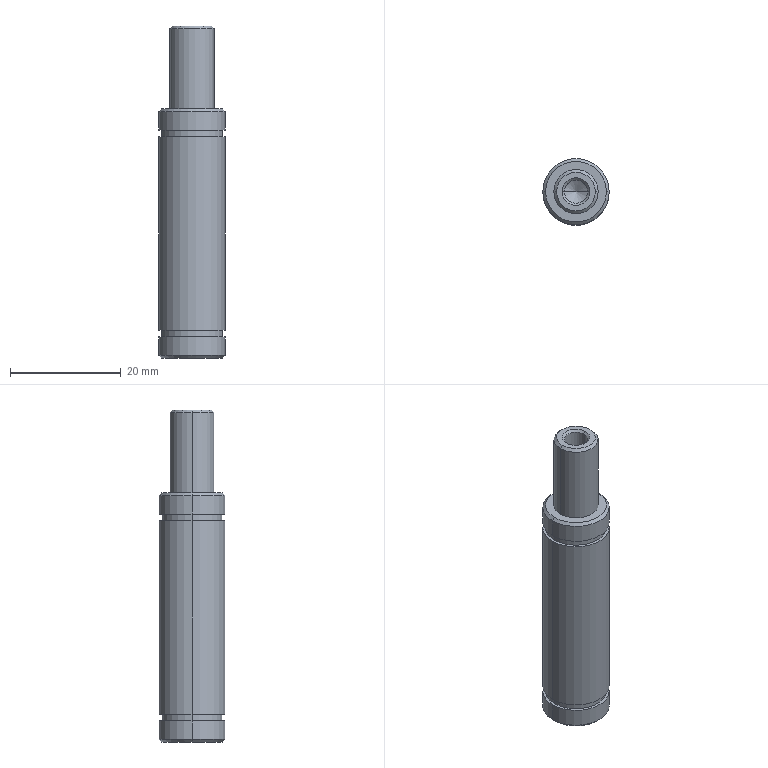Component | SolidWorks | GluePaperFeedingTensioningWheelAssembly-1_YX-04-118GluePaperFeedingTensioningWheelAxis-1 | 1 solid | 31 faces | box 12 x 12 x 60 mm | volume 5606 mm3 | cylinder 14 | cone 10 | plane 7 | commonest cylinder face diameters 12 x6 11 x4 8 x2 4.2 x2 | material 45#Steel
build123d program:
from build123d import *


with BuildPart() as part:
    # Sketch1 → Revolve1 (revolve)
    with BuildSketch(Plane.XY, mode=Mode.PRIVATE) as revolve1_sk:
        Polygon((12.6, 2.1), (13.862, 0), (60, 0), (60, 5.5), (59.5, 6), (56.2, 6), (56.2, 5.5), (55, 5.5), (55, 6), (20, 6), (20, 5.5), (18.8, 5.5), (18.8, 6), (15.5, 6), (15, 5.5), (15, 4), (0.5, 4), (0, 3.5), (0, 2.5), (0.4, 2.1), align=None)
    revolve(revolve1_sk.sketch.rotate(Axis((0, 0, 0), (1, 0, 0)), 270), axis=Axis((0, 0, 0), (1, 0, 0)))


solid = part.part

# Placed as in the assembly
solid = solid.moved(Location((16.603, 20.762, 174), (0, 90, 0)))
STEP:
#1=CARTESIAN_POINT('',(0.7363,0.8174,6.835));
#2=VERTEX_POINT('',#1);
#3=CARTESIAN_POINT('',(0.571,0.8174,6.835));
#4=VERTEX_POINT('',#3);
#5=CARTESIAN_POINT('',(0.6537,0.8174,6.835));
#6=DIRECTION('',(-0.,0.,-1.));
#7=DIRECTION('',(-1.,0.,0.));
#8=AXIS2_PLACEMENT_3D('',#5,#6,#7);
#9=CIRCLE('',#8,0.08268);
#10=EDGE_CURVE('',#2,#4,#9,.T.);
#11=ORIENTED_EDGE('',*,*,#10,.T.);
#12=CARTESIAN_POINT('',(0.5552,0.8174,6.85));
#13=VERTEX_POINT('',#12);
#14=CARTESIAN_POINT('',(0.5552,0.8174,6.85));
#15=DIRECTION('',(-0.7071,0.,0.7071));
#16=VECTOR('',#15,39.37);
#17=LINE('',#14,#16);
#18=EDGE_CURVE('',#4,#13,#17,.T.);
#19=ORIENTED_EDGE('',*,*,#18,.T.);
#20=CARTESIAN_POINT('',(0.7521,0.8174,6.85));
#21=VERTEX_POINT('',#20);
#22=CARTESIAN_POINT('',(0.6537,0.8174,6.85));
#23=DIRECTION('',(-0.,0.,-1.));
#24=DIRECTION('',(-1.,0.,0.));
#25=AXIS2_PLACEMENT_3D('',#22,#23,#24);
#26=CIRCLE('',#25,0.09843);
#27=EDGE_CURVE('',#21,#13,#26,.T.);
#28=ORIENTED_EDGE('',*,*,#27,.F.);
#29=CARTESIAN_POINT('',(0.7521,0.8174,6.85));
#30=DIRECTION('',(0.7071,0.,0.7071));
#31=VECTOR('',#30,39.37);
#32=LINE('',#29,#31);
#33=EDGE_CURVE('',#2,#21,#32,.T.);
#34=ORIENTED_EDGE('',*,*,#33,.F.);
#35=EDGE_LOOP('',(#11,#19,#28,#34));
#36=FACE_OUTER_BOUND('',#35,.T.);
#37=CARTESIAN_POINT('',(0.6537,0.8174,6.85));
#38=DIRECTION('',(0.,-0.,1.));
#39=DIRECTION('',(1.,0.,0.));
#40=AXIS2_PLACEMENT_3D('',#37,#38,#39);
#41=CONICAL_SURFACE('',#40,0.09843,0.7854);
#42=ADVANCED_FACE('',(#36),#41,.F.);
#43=CARTESIAN_POINT('',(0.5159,0.8174,6.85));
#44=VERTEX_POINT('',#43);
#45=CARTESIAN_POINT('',(0.7914,0.8174,6.85));
#46=VERTEX_POINT('',#45);
#47=CARTESIAN_POINT('',(0.6537,0.8174,6.85));
#48=DIRECTION('',(-0.,0.,-1.));
#49=DIRECTION('',(-1.,0.,0.));
#50=AXIS2_PLACEMENT_3D('',#47,#48,#49);
#51=CIRCLE('',#50,0.1378);
#52=EDGE_CURVE('',#44,#46,#51,.T.);
#53=ORIENTED_EDGE('',*,*,#52,.T.);
#54=CARTESIAN_POINT('',(0.8111,0.8174,6.831));
#55=VERTEX_POINT('',#54);
#56=CARTESIAN_POINT('',(0.8111,0.8174,6.831));
#57=DIRECTION('',(0.7071,0.,-0.7071));
#58=VECTOR('',#57,39.37);
#59=LINE('',#56,#58);
#60=EDGE_CURVE('',#46,#55,#59,.T.);
#61=ORIENTED_EDGE('',*,*,#60,.T.);
#62=CARTESIAN_POINT('',(0.4962,0.8174,6.831));
#63=VERTEX_POINT('',#62);
#64=CARTESIAN_POINT('',(0.6537,0.8174,6.831));
#65=DIRECTION('',(-0.,0.,-1.));
#66=DIRECTION('',(-1.,0.,0.));
#67=AXIS2_PLACEMENT_3D('',#64,#65,#66);
#68=CIRCLE('',#67,0.1575);
#69=EDGE_CURVE('',#63,#55,#68,.T.);
#70=ORIENTED_EDGE('',*,*,#69,.F.);
#71=CARTESIAN_POINT('',(0.4962,0.8174,6.831));
#72=DIRECTION('',(-0.7071,-0.,-0.7071));
#73=VECTOR('',#72,39.37);
#74=LINE('',#71,#73);
#75=EDGE_CURVE('',#44,#63,#74,.T.);
#76=ORIENTED_EDGE('',*,*,#75,.F.);
#77=EDGE_LOOP('',(#53,#61,#70,#76));
#78=FACE_OUTER_BOUND('',#77,.T.);
#79=CARTESIAN_POINT('',(0.6537,0.8174,6.831));
#80=DIRECTION('',(-0.,0.,-1.));
#81=DIRECTION('',(-1.,0.,0.));
#82=AXIS2_PLACEMENT_3D('',#79,#80,#81);
#83=CONICAL_SURFACE('',#82,0.1575,0.7854);
#84=ADVANCED_FACE('',(#78),#83,.T.);
#85=ORIENTED_EDGE('',*,*,#69,.T.);
#86=CARTESIAN_POINT('',(0.8111,0.8174,6.26));
#87=VERTEX_POINT('',#86);
#88=CARTESIAN_POINT('',(0.8111,0.8174,6.85));
#89=DIRECTION('',(-0.,0.,-1.));
#90=VECTOR('',#89,39.37);
#91=LINE('',#88,#90);
#92=EDGE_CURVE('',#55,#87,#91,.T.);
#93=ORIENTED_EDGE('',*,*,#92,.T.);
#94=CARTESIAN_POINT('',(0.4962,0.8174,6.26));
#95=VERTEX_POINT('',#94);
#96=CARTESIAN_POINT('',(0.6537,0.8174,6.26));
#97=DIRECTION('',(-0.,0.,-1.));
#98=DIRECTION('',(-1.,0.,0.));
#99=AXIS2_PLACEMENT_3D('',#96,#97,#98);
#100=CIRCLE('',#99,0.1575);
#101=EDGE_CURVE('',#95,#87,#100,.T.);
#102=ORIENTED_EDGE('',*,*,#101,.F.);
#103=CARTESIAN_POINT('',(0.4962,0.8174,6.85));
#104=DIRECTION('',(-0.,0.,-1.));
#105=VECTOR('',#104,39.37);
#106=LINE('',#103,#105);
#107=EDGE_CURVE('',#63,#95,#106,.T.);
#108=ORIENTED_EDGE('',*,*,#107,.F.);
#109=EDGE_LOOP('',(#85,#93,#102,#108));
#110=FACE_OUTER_BOUND('',#109,.T.);
#111=CARTESIAN_POINT('',(0.6537,0.8174,6.85));
#112=DIRECTION('',(-0.,0.,-1.));
#113=DIRECTION('',(-1.,0.,0.));
#114=AXIS2_PLACEMENT_3D('',#111,#112,#113);
#115=CYLINDRICAL_SURFACE('',#114,0.1575);
#116=ADVANCED_FACE('',(#110),#115,.T.);
#117=CARTESIAN_POINT('',(0.4371,0.8174,6.26));
#118=VERTEX_POINT('',#117);
#119=CARTESIAN_POINT('',(0.8702,0.8174,6.26));
#120=VERTEX_POINT('',#119);
#121=CARTESIAN_POINT('',(0.6537,0.8174,6.26));
#122=DIRECTION('',(-0.,0.,-1.));
#123=DIRECTION('',(-1.,0.,0.));
#124=AXIS2_PLACEMENT_3D('',#121,#122,#123);
#125=CIRCLE('',#124,0.2165);
#126=EDGE_CURVE('',#118,#120,#125,.T.);
#127=ORIENTED_EDGE('',*,*,#126,.T.);
#128=CARTESIAN_POINT('',(0.8899,0.8174,6.24));
#129=VERTEX_POINT('',#128);
#130=CARTESIAN_POINT('',(0.8899,0.8174,6.24));
#131=DIRECTION('',(0.7071,0.,-0.7071));
#132=VECTOR('',#131,39.37);
#133=LINE('',#130,#132);
#134=EDGE_CURVE('',#120,#129,#133,.T.);
#135=ORIENTED_EDGE('',*,*,#134,.T.);
#136=CARTESIAN_POINT('',(0.4174,0.8174,6.24));
#137=VERTEX_POINT('',#136);
#138=CARTESIAN_POINT('',(0.6537,0.8174,6.24));
#139=DIRECTION('',(-0.,0.,-1.));
#140=DIRECTION('',(-1.,0.,0.));
#141=AXIS2_PLACEMENT_3D('',#138,#139,#140);
#142=CIRCLE('',#141,0.2362);
#143=EDGE_CURVE('',#137,#129,#142,.T.);
#144=ORIENTED_EDGE('',*,*,#143,.F.);
#145=CARTESIAN_POINT('',(0.4174,0.8174,6.24));
#146=DIRECTION('',(-0.7071,-0.,-0.7071));
#147=VECTOR('',#146,39.37);
#148=LINE('',#145,#147);
#149=EDGE_CURVE('',#118,#137,#148,.T.);
#150=ORIENTED_EDGE('',*,*,#149,.F.);
#151=EDGE_LOOP('',(#127,#135,#144,#150));
#152=FACE_OUTER_BOUND('',#151,.T.);
#153=CARTESIAN_POINT('',(0.6537,0.8174,6.24));
#154=DIRECTION('',(-0.,0.,-1.));
#155=DIRECTION('',(-1.,0.,0.));
#156=AXIS2_PLACEMENT_3D('',#153,#154,#155);
#157=CONICAL_SURFACE('',#156,0.2362,0.7854);
#158=ADVANCED_FACE('',(#152),#157,.T.);
#159=ORIENTED_EDGE('',*,*,#143,.T.);
#160=CARTESIAN_POINT('',(0.8899,0.8174,6.11));
#161=VERTEX_POINT('',#160);
#162=CARTESIAN_POINT('',(0.8899,0.8174,6.85));
#163=DIRECTION('',(-0.,0.,-1.));
#164=VECTOR('',#163,39.37);
#165=LINE('',#162,#164);
#166=EDGE_CURVE('',#129,#161,#165,.T.);
#167=ORIENTED_EDGE('',*,*,#166,.T.);
#168=CARTESIAN_POINT('',(0.4174,0.8174,6.11));
#169=VERTEX_POINT('',#168);
#170=CARTESIAN_POINT('',(0.6537,0.8174,6.11));
#171=DIRECTION('',(-0.,0.,-1.));
#172=DIRECTION('',(-1.,0.,0.));
#173=AXIS2_PLACEMENT_3D('',#170,#171,#172);
#174=CIRCLE('',#173,0.2362);
#175=EDGE_CURVE('',#169,#161,#174,.T.);
#176=ORIENTED_EDGE('',*,*,#175,.F.);
#177=CARTESIAN_POINT('',(0.4174,0.8174,6.85));
#178=DIRECTION('',(-0.,0.,-1.));
#179=VECTOR('',#178,39.37);
#180=LINE('',#177,#179);
#181=EDGE_CURVE('',#137,#169,#180,.T.);
#182=ORIENTED_EDGE('',*,*,#181,.F.);
#183=EDGE_LOOP('',(#159,#167,#176,#182));
#184=FACE_OUTER_BOUND('',#183,.T.);
#185=CARTESIAN_POINT('',(0.6537,0.8174,6.85));
#186=DIRECTION('',(-0.,0.,-1.));
#187=DIRECTION('',(-1.,0.,0.));
#188=AXIS2_PLACEMENT_3D('',#185,#186,#187);
#189=CYLINDRICAL_SURFACE('',#188,0.2362);
#190=ADVANCED_FACE('',(#184),#189,.T.);
#191=CARTESIAN_POINT('',(0.4371,0.8174,6.11));
#192=VERTEX_POINT('',#191);
#193=CARTESIAN_POINT('',(0.8702,0.8174,6.11));
#194=VERTEX_POINT('',#193);
#195=CARTESIAN_POINT('',(0.6537,0.8174,6.11));
#196=DIRECTION('',(-0.,0.,-1.));
#197=DIRECTION('',(-1.,0.,0.));
#198=AXIS2_PLACEMENT_3D('',#195,#196,#197);
#199=CIRCLE('',#198,0.2165);
#200=EDGE_CURVE('',#192,#194,#199,.T.);
#201=ORIENTED_EDGE('',*,*,#200,.T.);
#202=CARTESIAN_POINT('',(0.8702,0.8174,6.063));
#203=VERTEX_POINT('',#202);
#204=CARTESIAN_POINT('',(0.8702,0.8174,6.85));
#205=DIRECTION('',(-0.,0.,-1.));
#206=VECTOR('',#205,39.37);
#207=LINE('',#204,#206);
#208=EDGE_CURVE('',#194,#203,#207,.T.);
#209=ORIENTED_EDGE('',*,*,#208,.T.);
#210=CARTESIAN_POINT('',(0.4371,0.8174,6.063));
#211=VERTEX_POINT('',#210);
#212=CARTESIAN_POINT('',(0.6537,0.8174,6.063));
#213=DIRECTION('',(-0.,0.,-1.));
#214=DIRECTION('',(-1.,0.,0.));
#215=AXIS2_PLACEMENT_3D('',#212,#213,#214);
#216=CIRCLE('',#215,0.2165);
#217=EDGE_CURVE('',#211,#203,#216,.T.);
#218=ORIENTED_EDGE('',*,*,#217,.F.);
#219=CARTESIAN_POINT('',(0.4371,0.8174,6.85));
#220=DIRECTION('',(-0.,0.,-1.));
#221=VECTOR('',#220,39.37);
#222=LINE('',#219,#221);
#223=EDGE_CURVE('',#192,#211,#222,.T.);
#224=ORIENTED_EDGE('',*,*,#223,.F.);
#225=EDGE_LOOP('',(#201,#209,#218,#224));
#226=FACE_OUTER_BOUND('',#225,.T.);
#227=CARTESIAN_POINT('',(0.6537,0.8174,6.85));
#228=DIRECTION('',(-0.,0.,-1.));
#229=DIRECTION('',(-1.,0.,0.));
#230=AXIS2_PLACEMENT_3D('',#227,#228,#229);
#231=CYLINDRICAL_SURFACE('',#230,0.2165);
#232=ADVANCED_FACE('',(#226),#231,.T.);
#233=CARTESIAN_POINT('',(0.4174,0.8174,6.063));
#234=VERTEX_POINT('',#233);
#235=CARTESIAN_POINT('',(0.8899,0.8174,6.063));
#236=VERTEX_POINT('',#235);
#237=CARTESIAN_POINT('',(0.6537,0.8174,6.063));
#238=DIRECTION('',(-0.,0.,-1.));
#239=DIRECTION('',(-1.,0.,0.));
#240=AXIS2_PLACEMENT_3D('',#237,#238,#239);
#241=CIRCLE('',#240,0.2362);
#242=EDGE_CURVE('',#234,#236,#241,.T.);
#243=ORIENTED_EDGE('',*,*,#242,.T.);
#244=CARTESIAN_POINT('',(0.8899,0.8174,4.685));
#245=VERTEX_POINT('',#244);
#246=CARTESIAN_POINT('',(0.8899,0.8174,6.85));
#247=DIRECTION('',(-0.,0.,-1.));
#248=VECTOR('',#247,39.37);
#249=LINE('',#246,#248);
#250=EDGE_CURVE('',#236,#245,#249,.T.);
#251=ORIENTED_EDGE('',*,*,#250,.T.);
#252=CARTESIAN_POINT('',(0.4174,0.8174,4.685));
#253=VERTEX_POINT('',#252);
#254=CARTESIAN_POINT('',(0.6537,0.8174,4.685));
#255=DIRECTION('',(-0.,0.,-1.));
#256=DIRECTION('',(-1.,0.,0.));
#257=AXIS2_PLACEMENT_3D('',#254,#255,#256);
#258=CIRCLE('',#257,0.2362);
#259=EDGE_CURVE('',#253,#245,#258,.T.);
#260=ORIENTED_EDGE('',*,*,#259,.F.);
#261=CARTESIAN_POINT('',(0.4174,0.8174,6.85));
#262=DIRECTION('',(-0.,0.,-1.));
#263=VECTOR('',#262,39.37);
#264=LINE('',#261,#263);
#265=EDGE_CURVE('',#234,#253,#264,.T.);
#266=ORIENTED_EDGE('',*,*,#265,.F.);
#267=EDGE_LOOP('',(#243,#251,#260,#266));
#268=FACE_OUTER_BOUND('',#267,.T.);
#269=CARTESIAN_POINT('',(0.6537,0.8174,6.85));
#270=DIRECTION('',(-0.,0.,-1.));
#271=DIRECTION('',(-1.,0.,0.));
#272=AXIS2_PLACEMENT_3D('',#269,#270,#271);
#273=CYLINDRICAL_SURFACE('',#272,0.2362);
#274=ADVANCED_FACE('',(#268),#273,.T.);
#275=CARTESIAN_POINT('',(0.4371,0.8174,4.685));
#276=VERTEX_POINT('',#275);
#277=CARTESIAN_POINT('',(0.8702,0.8174,4.685));
#278=VERTEX_POINT('',#277);
#279=CARTESIAN_POINT('',(0.6537,0.8174,4.685));
#280=DIRECTION('',(-0.,0.,-1.));
#281=DIRECTION('',(-1.,0.,0.));
#282=AXIS2_PLACEMENT_3D('',#279,#280,#281);
#283=CIRCLE('',#282,0.2165);
#284=EDGE_CURVE('',#276,#278,#283,.T.);
#285=ORIENTED_EDGE('',*,*,#284,.T.);
#286=CARTESIAN_POINT('',(0.8702,0.8174,4.638));
#287=VERTEX_POINT('',#286);
#288=CARTESIAN_POINT('',(0.8702,0.8174,6.85));
#289=DIRECTION('',(-0.,0.,-1.));
#290=VECTOR('',#289,39.37);
#291=LINE('',#288,#290);
#292=EDGE_CURVE('',#278,#287,#291,.T.);
#293=ORIENTED_EDGE('',*,*,#292,.T.);
#294=CARTESIAN_POINT('',(0.4371,0.8174,4.638));
#295=VERTEX_POINT('',#294);
#296=CARTESIAN_POINT('',(0.6537,0.8174,4.638));
#297=DIRECTION('',(-0.,0.,-1.));
#298=DIRECTION('',(-1.,0.,0.));
#299=AXIS2_PLACEMENT_3D('',#296,#297,#298);
#300=CIRCLE('',#299,0.2165);
#301=EDGE_CURVE('',#295,#287,#300,.T.);
#302=ORIENTED_EDGE('',*,*,#301,.F.);
#303=CARTESIAN_POINT('',(0.4371,0.8174,6.85));
#304=DIRECTION('',(-0.,0.,-1.));
#305=VECTOR('',#304,39.37);
#306=LINE('',#303,#305);
#307=EDGE_CURVE('',#276,#295,#306,.T.);
#308=ORIENTED_EDGE('',*,*,#307,.F.);
#309=EDGE_LOOP('',(#285,#293,#302,#308));
#310=FACE_OUTER_BOUND('',#309,.T.);
#311=CARTESIAN_POINT('',(0.6537,0.8174,6.85));
#312=DIRECTION('',(-0.,0.,-1.));
#313=DIRECTION('',(-1.,0.,0.));
#314=AXIS2_PLACEMENT_3D('',#311,#312,#313);
#315=CYLINDRICAL_SURFACE('',#314,0.2165);
#316=ADVANCED_FACE('',(#310),#315,.T.);
#317=CARTESIAN_POINT('',(0.4174,0.8174,4.638));
#318=VERTEX_POINT('',#317);
#319=CARTESIAN_POINT('',(0.8899,0.8174,4.638));
#320=VERTEX_POINT('',#319);
#321=CARTESIAN_POINT('',(0.6537,0.8174,4.638));
#322=DIRECTION('',(-0.,0.,-1.));
#323=DIRECTION('',(-1.,0.,0.));
#324=AXIS2_PLACEMENT_3D('',#321,#322,#323);
#325=CIRCLE('',#324,0.2362);
#326=EDGE_CURVE('',#318,#320,#325,.T.);
#327=ORIENTED_EDGE('',*,*,#326,.T.);
#328=CARTESIAN_POINT('',(0.8899,0.8174,4.508));
#329=VERTEX_POINT('',#328);
#330=CARTESIAN_POINT('',(0.8899,0.8174,6.85));
#331=DIRECTION('',(-0.,0.,-1.));
#332=VECTOR('',#331,39.37);
#333=LINE('',#330,#332);
#334=EDGE_CURVE('',#320,#329,#333,.T.);
#335=ORIENTED_EDGE('',*,*,#334,.T.);
#336=CARTESIAN_POINT('',(0.4174,0.8174,4.508));
#337=VERTEX_POINT('',#336);
#338=CARTESIAN_POINT('',(0.6537,0.8174,4.508));
#339=DIRECTION('',(-0.,0.,-1.));
#340=DIRECTION('',(-1.,0.,0.));
#341=AXIS2_PLACEMENT_3D('',#338,#339,#340);
#342=CIRCLE('',#341,0.2362);
#343=EDGE_CURVE('',#337,#329,#342,.T.);
#344=ORIENTED_EDGE('',*,*,#343,.F.);
#345=CARTESIAN_POINT('',(0.4174,0.8174,6.85));
#346=DIRECTION('',(-0.,0.,-1.));
#347=VECTOR('',#346,39.37);
#348=LINE('',#345,#347);
#349=EDGE_CURVE('',#318,#337,#348,.T.);
#350=ORIENTED_EDGE('',*,*,#349,.F.);
#351=EDGE_LOOP('',(#327,#335,#344,#350));
#352=FACE_OUTER_BOUND('',#351,.T.);
#353=CARTESIAN_POINT('',(0.6537,0.8174,6.85));
#354=DIRECTION('',(-0.,0.,-1.));
#355=DIRECTION('',(-1.,0.,0.));
#356=AXIS2_PLACEMENT_3D('',#353,#354,#355);
#357=CYLINDRICAL_SURFACE('',#356,0.2362);
#358=ADVANCED_FACE('',(#352),#357,.T.);
#359=CARTESIAN_POINT('',(0.4371,0.8174,4.488));
#360=VERTEX_POINT('',#359);
#361=CARTESIAN_POINT('',(0.8702,0.8174,4.488));
#362=VERTEX_POINT('',#361);
#363=CARTESIAN_POINT('',(0.6537,0.8174,4.488));
#364=DIRECTION('',(-0.,0.,-1.));
#365=DIRECTION('',(-1.,0.,0.));
#366=AXIS2_PLACEMENT_3D('',#363,#364,#365);
#367=CIRCLE('',#366,0.2165);
#368=EDGE_CURVE('',#360,#362,#367,.T.);
#369=ORIENTED_EDGE('',*,*,#368,.F.);
#370=CARTESIAN_POINT('',(0.4371,0.8174,4.488));
#371=DIRECTION('',(-0.7071,0.,0.7071));
#372=VECTOR('',#371,39.37);
#373=LINE('',#370,#372);
#374=EDGE_CURVE('',#360,#337,#373,.T.);
#375=ORIENTED_EDGE('',*,*,#374,.T.);
#376=ORIENTED_EDGE('',*,*,#343,.T.);
#377=CARTESIAN_POINT('',(0.8702,0.8174,4.488));
#378=DIRECTION('',(0.7071,0.,0.7071));
#379=VECTOR('',#378,39.37);
#380=LINE('',#377,#379);
#381=EDGE_CURVE('',#362,#329,#380,.T.);
#382=ORIENTED_EDGE('',*,*,#381,.F.);
#383=EDGE_LOOP('',(#369,#375,#376,#382));
#384=FACE_OUTER_BOUND('',#383,.T.);
#385=CARTESIAN_POINT('',(0.6537,0.8174,4.488));
#386=DIRECTION('',(0.,-0.,1.));
#387=DIRECTION('',(1.,0.,0.));
#388=AXIS2_PLACEMENT_3D('',#385,#386,#387);
#389=CONICAL_SURFACE('',#388,0.2165,0.7854);
#390=ADVANCED_FACE('',(#384),#389,.T.);
#391=CARTESIAN_POINT('',(0.6537,0.8174,6.305));
#392=VERTEX_POINT('',#391);
#393=CARTESIAN_POINT('',(0.7363,0.8174,6.354));
#394=VERTEX_POINT('',#393);
#395=CARTESIAN_POINT('',(0.7363,0.8174,6.354));
#396=DIRECTION('',(0.8572,0.,0.515));
#397=VECTOR('',#396,39.37);
#398=LINE('',#395,#397);
#399=EDGE_CURVE('',#392,#394,#398,.T.);
#400=ORIENTED_EDGE('',*,*,#399,.F.);
#401=CARTESIAN_POINT('',(0.571,0.8174,6.354));
#402=VERTEX_POINT('',#401);
#403=CARTESIAN_POINT('',(0.571,0.8174,6.354));
#404=DIRECTION('',(-0.8572,0.,0.515));
#405=VECTOR('',#404,39.37);
#406=LINE('',#403,#405);
#407=EDGE_CURVE('',#392,#402,#406,.T.);
#408=ORIENTED_EDGE('',*,*,#407,.T.);
#409=CARTESIAN_POINT('',(0.6537,0.8174,6.354));
#410=DIRECTION('',(-0.,0.,-1.));
#411=DIRECTION('',(-1.,0.,0.));
#412=AXIS2_PLACEMENT_3D('',#409,#410,#411);
#413=CIRCLE('',#412,0.08268);
#414=EDGE_CURVE('',#394,#402,#413,.T.);
#415=ORIENTED_EDGE('',*,*,#414,.F.);
#416=EDGE_LOOP('',(#400,#408,#415));
#417=FACE_OUTER_BOUND('',#416,.T.);
#418=CARTESIAN_POINT('',(0.6537,0.8174,6.354));
#419=DIRECTION('',(0.,-0.,1.));
#420=DIRECTION('',(1.,0.,0.));
#421=AXIS2_PLACEMENT_3D('',#418,#419,#420);
#422=CONICAL_SURFACE('',#421,0.08268,1.03);
#423=ADVANCED_FACE('',(#417),#422,.F.);
#424=ORIENTED_EDGE('',*,*,#10,.F.);
#425=CARTESIAN_POINT('',(0.7363,0.8174,6.85));
#426=DIRECTION('',(-0.,0.,-1.));
#427=VECTOR('',#426,39.37);
#428=LINE('',#425,#427);
#429=EDGE_CURVE('',#2,#394,#428,.T.);
#430=ORIENTED_EDGE('',*,*,#429,.T.);
#431=ORIENTED_EDGE('',*,*,#414,.T.);
#432=CARTESIAN_POINT('',(0.571,0.8174,6.85));
#433=DIRECTION('',(-0.,0.,-1.));
#434=VECTOR('',#433,39.37);
#435=LINE('',#432,#434);
#436=EDGE_CURVE('',#4,#402,#435,.T.);
#437=ORIENTED_EDGE('',*,*,#436,.F.);
#438=EDGE_LOOP('',(#424,#430,#431,#437));
#439=FACE_OUTER_BOUND('',#438,.T.);
#440=CARTESIAN_POINT('',(0.6537,0.8174,6.85));
#441=DIRECTION('',(-0.,0.,-1.));
#442=DIRECTION('',(-1.,0.,0.));
#443=AXIS2_PLACEMENT_3D('',#440,#441,#442);
#444=CYLINDRICAL_SURFACE('',#443,0.08268);
#445=ADVANCED_FACE('',(#439),#444,.F.);
#446=ORIENTED_EDGE('',*,*,#429,.F.);
#447=CARTESIAN_POINT('',(0.6537,0.8174,6.835));
#448=DIRECTION('',(-0.,0.,-1.));
#449=DIRECTION('',(-1.,0.,0.));
#450=AXIS2_PLACEMENT_3D('',#447,#448,#449);
#451=CIRCLE('',#450,0.08268);
#452=EDGE_CURVE('',#4,#2,#451,.T.);
#453=ORIENTED_EDGE('',*,*,#452,.F.);
#454=ORIENTED_EDGE('',*,*,#436,.T.);
#455=CARTESIAN_POINT('',(0.6537,0.8174,6.354));
#456=DIRECTION('',(-0.,0.,-1.));
#457=DIRECTION('',(-1.,0.,0.));
#458=AXIS2_PLACEMENT_3D('',#455,#456,#457);
#459=CIRCLE('',#458,0.08268);
#460=EDGE_CURVE('',#402,#394,#459,.T.);
#461=ORIENTED_EDGE('',*,*,#460,.T.);
#462=EDGE_LOOP('',(#446,#453,#454,#461));
#463=FACE_OUTER_BOUND('',#462,.T.);
#464=CARTESIAN_POINT('',(0.6537,0.8174,6.85));
#465=DIRECTION('',(-0.,0.,-1.));
#466=DIRECTION('',(-1.,0.,0.));
#467=AXIS2_PLACEMENT_3D('',#464,#465,#466);
#468=CYLINDRICAL_SURFACE('',#467,0.08268);
#469=ADVANCED_FACE('',(#463),#468,.F.);
#470=ORIENTED_EDGE('',*,*,#407,.F.);
#471=ORIENTED_EDGE('',*,*,#399,.T.);
#472=ORIENTED_EDGE('',*,*,#460,.F.);
#473=EDGE_LOOP('',(#470,#471,#472));
#474=FACE_OUTER_BOUND('',#473,.T.);
#475=CARTESIAN_POINT('',(0.6537,0.8174,6.354));
#476=DIRECTION('',(0.,-0.,1.));
#477=DIRECTION('',(1.,0.,0.));
#478=AXIS2_PLACEMENT_3D('',#475,#476,#477);
#479=CONICAL_SURFACE('',#478,0.08268,1.03);
#480=ADVANCED_FACE('',(#474),#479,.F.);
#481=CARTESIAN_POINT('',(0.6537,0.8174,4.488));
#482=DIRECTION('',(-0.,0.,-1.));
#483=DIRECTION('',(-1.,0.,0.));
#484=AXIS2_PLACEMENT_3D('',#481,#482,#483);
#485=CIRCLE('',#484,0.2165);
#486=EDGE_CURVE('',#362,#360,#485,.T.);
#487=ORIENTED_EDGE('',*,*,#486,.T.);
#488=ORIENTED_EDGE('',*,*,#368,.T.);
#489=EDGE_LOOP('',(#487,#488));
#490=FACE_OUTER_BOUND('',#489,.T.);
#491=CARTESIAN_POINT('',(0.6537,0.8174,4.488));
#492=DIRECTION('',(-0.,0.,-1.));
#493=DIRECTION('',(-1.,-0.,0.));
#494=AXIS2_PLACEMENT_3D('',#491,#492,#493);
#495=PLANE('',#494);
#496=ADVANCED_FACE('',(#490),#495,.T.);
#497=ORIENTED_EDGE('',*,*,#374,.F.);
#498=ORIENTED_EDGE('',*,*,#486,.F.);
#499=ORIENTED_EDGE('',*,*,#381,.T.);
#500=CARTESIAN_POINT('',(0.6537,0.8174,4.508));
#501=DIRECTION('',(-0.,0.,-1.));
#502=DIRECTION('',(-1.,0.,0.));
#503=AXIS2_PLACEMENT_3D('',#500,#501,#502);
#504=CIRCLE('',#503,0.2362);
#505=EDGE_CURVE('',#329,#337,#504,.T.);
#506=ORIENTED_EDGE('',*,*,#505,.T.);
#507=EDGE_LOOP('',(#497,#498,#499,#506));
#508=FACE_OUTER_BOUND('',#507,.T.);
#509=CARTESIAN_POINT('',(0.6537,0.8174,4.488));
#510=DIRECTION('',(0.,-0.,1.));
#511=DIRECTION('',(1.,0.,0.));
#512=AXIS2_PLACEMENT_3D('',#509,#510,#511);
#513=CONICAL_SURFACE('',#512,0.2165,0.7854);
#514=ADVANCED_FACE('',(#508),#513,.T.);
#515=ORIENTED_EDGE('',*,*,#334,.F.);
#516=CARTESIAN_POINT('',(0.6537,0.8174,4.638));
#517=DIRECTION('',(-0.,0.,-1.));
#518=DIRECTION('',(-1.,0.,0.));
#519=AXIS2_PLACEMENT_3D('',#516,#517,#518);
#520=CIRCLE('',#519,0.2362);
#521=EDGE_CURVE('',#320,#318,#520,.T.);
#522=ORIENTED_EDGE('',*,*,#521,.T.);
#523=ORIENTED_EDGE('',*,*,#349,.T.);
#524=ORIENTED_EDGE('',*,*,#505,.F.);
#525=EDGE_LOOP('',(#515,#522,#523,#524));
#526=FACE_OUTER_BOUND('',#525,.T.);
#527=CARTESIAN_POINT('',(0.6537,0.8174,6.85));
#528=DIRECTION('',(-0.,0.,-1.));
#529=DIRECTION('',(-1.,0.,0.));
#530=AXIS2_PLACEMENT_3D('',#527,#528,#529);
#531=CYLINDRICAL_SURFACE('',#530,0.2362);
#532=ADVANCED_FACE('',(#526),#531,.T.);
#533=ORIENTED_EDGE('',*,*,#301,.T.);
#534=CARTESIAN_POINT('',(0.6537,0.8174,4.638));
#535=DIRECTION('',(-0.,0.,-1.));
#536=DIRECTION('',(-1.,0.,0.));
#537=AXIS2_PLACEMENT_3D('',#534,#535,#536);
#538=CIRCLE('',#537,0.2165);
#539=EDGE_CURVE('',#287,#295,#538,.T.);
#540=ORIENTED_EDGE('',*,*,#539,.T.);
#541=EDGE_LOOP('',(#533,#540));
#542=FACE_BOUND('',#541,.T.);
#543=ORIENTED_EDGE('',*,*,#326,.F.);
#544=ORIENTED_EDGE('',*,*,#521,.F.);
#545=EDGE_LOOP('',(#543,#544));
#546=FACE_OUTER_BOUND('',#545,.T.);
#547=CARTESIAN_POINT('',(0.6537,1.054,4.638));
#548=DIRECTION('',(0.,-0.,1.));
#549=DIRECTION('',(1.,0.,-0.));
#550=AXIS2_PLACEMENT_3D('',#547,#548,#549);
#551=PLANE('',#550);
#552=ADVANCED_FACE('',(#542,#546),#551,.T.);
#553=ORIENTED_EDGE('',*,*,#292,.F.);
#554=CARTESIAN_POINT('',(0.6537,0.8174,4.685));
#555=DIRECTION('',(-0.,0.,-1.));
#556=DIRECTION('',(-1.,0.,0.));
#557=AXIS2_PLACEMENT_3D('',#554,#555,#556);
#558=CIRCLE('',#557,0.2165);
#559=EDGE_CURVE('',#278,#276,#558,.T.);
#560=ORIENTED_EDGE('',*,*,#559,.T.);
#561=ORIENTED_EDGE('',*,*,#307,.T.);
#562=ORIENTED_EDGE('',*,*,#539,.F.);
#563=EDGE_LOOP('',(#553,#560,#561,#562));
#564=FACE_OUTER_BOUND('',#563,.T.);
#565=CARTESIAN_POINT('',(0.6537,0.8174,6.85));
#566=DIRECTION('',(-0.,0.,-1.));
#567=DIRECTION('',(-1.,0.,0.));
#568=AXIS2_PLACEMENT_3D('',#565,#566,#567);
#569=CYLINDRICAL_SURFACE('',#568,0.2165);
#570=ADVANCED_FACE('',(#564),#569,.T.);
#571=ORIENTED_EDGE('',*,*,#259,.T.);
#572=CARTESIAN_POINT('',(0.6537,0.8174,4.685));
#573=DIRECTION('',(-0.,0.,-1.));
#574=DIRECTION('',(-1.,0.,0.));
#575=AXIS2_PLACEMENT_3D('',#572,#573,#574);
#576=CIRCLE('',#575,0.2362);
#577=EDGE_CURVE('',#245,#253,#576,.T.);
#578=ORIENTED_EDGE('',*,*,#577,.T.);
#579=EDGE_LOOP('',(#571,#578));
#580=FACE_OUTER_BOUND('',#579,.T.);
#581=ORIENTED_EDGE('',*,*,#284,.F.);
#582=ORIENTED_EDGE('',*,*,#559,.F.);
#583=EDGE_LOOP('',(#581,#582));
#584=FACE_BOUND('',#583,.T.);
#585=CARTESIAN_POINT('',(0.6537,1.034,4.685));
#586=DIRECTION('',(-0.,0.,-1.));
#587=DIRECTION('',(-1.,-0.,0.));
#588=AXIS2_PLACEMENT_3D('',#585,#586,#587);
#589=PLANE('',#588);
#590=ADVANCED_FACE('',(#580,#584),#589,.T.);
#591=ORIENTED_EDGE('',*,*,#250,.F.);
#592=CARTESIAN_POINT('',(0.6537,0.8174,6.063));
#593=DIRECTION('',(-0.,0.,-1.));
#594=DIRECTION('',(-1.,0.,0.));
#595=AXIS2_PLACEMENT_3D('',#592,#593,#594);
#596=CIRCLE('',#595,0.2362);
#597=EDGE_CURVE('',#236,#234,#596,.T.);
#598=ORIENTED_EDGE('',*,*,#597,.T.);
#599=ORIENTED_EDGE('',*,*,#265,.T.);
#600=ORIENTED_EDGE('',*,*,#577,.F.);
#601=EDGE_LOOP('',(#591,#598,#599,#600));
#602=FACE_OUTER_BOUND('',#601,.T.);
#603=CARTESIAN_POINT('',(0.6537,0.8174,6.85));
#604=DIRECTION('',(-0.,0.,-1.));
#605=DIRECTION('',(-1.,0.,0.));
#606=AXIS2_PLACEMENT_3D('',#603,#604,#605);
#607=CYLINDRICAL_SURFACE('',#606,0.2362);
#608=ADVANCED_FACE('',(#602),#607,.T.);
#609=ORIENTED_EDGE('',*,*,#217,.T.);
#610=CARTESIAN_POINT('',(0.6537,0.8174,6.063));
#611=DIRECTION('',(-0.,0.,-1.));
#612=DIRECTION('',(-1.,0.,0.));
#613=AXIS2_PLACEMENT_3D('',#610,#611,#612);
#614=CIRCLE('',#613,0.2165);
#615=EDGE_CURVE('',#203,#211,#614,.T.);
#616=ORIENTED_EDGE('',*,*,#615,.T.);
#617=EDGE_LOOP('',(#609,#616));
#618=FACE_BOUND('',#617,.T.);
#619=ORIENTED_EDGE('',*,*,#242,.F.);
#620=ORIENTED_EDGE('',*,*,#597,.F.);
#621=EDGE_LOOP('',(#619,#620));
#622=FACE_OUTER_BOUND('',#621,.T.);
#623=CARTESIAN_POINT('',(0.6537,1.054,6.063));
#624=DIRECTION('',(0.,-0.,1.));
#625=DIRECTION('',(1.,0.,-0.));
#626=AXIS2_PLACEMENT_3D('',#623,#624,#625);
#627=PLANE('',#626);
#628=ADVANCED_FACE('',(#618,#622),#627,.T.);
#629=ORIENTED_EDGE('',*,*,#208,.F.);
#630=CARTESIAN_POINT('',(0.6537,0.8174,6.11));
#631=DIRECTION('',(-0.,0.,-1.));
#632=DIRECTION('',(-1.,0.,0.));
#633=AXIS2_PLACEMENT_3D('',#630,#631,#632);
#634=CIRCLE('',#633,0.2165);
#635=EDGE_CURVE('',#194,#192,#634,.T.);
#636=ORIENTED_EDGE('',*,*,#635,.T.);
#637=ORIENTED_EDGE('',*,*,#223,.T.);
#638=ORIENTED_EDGE('',*,*,#615,.F.);
#639=EDGE_LOOP('',(#629,#636,#637,#638));
#640=FACE_OUTER_BOUND('',#639,.T.);
#641=CARTESIAN_POINT('',(0.6537,0.8174,6.85));
#642=DIRECTION('',(-0.,0.,-1.));
#643=DIRECTION('',(-1.,0.,0.));
#644=AXIS2_PLACEMENT_3D('',#641,#642,#643);
#645=CYLINDRICAL_SURFACE('',#644,0.2165);
#646=ADVANCED_FACE('',(#640),#645,.T.);
#647=ORIENTED_EDGE('',*,*,#175,.T.);
#648=CARTESIAN_POINT('',(0.6537,0.8174,6.11));
#649=DIRECTION('',(-0.,0.,-1.));
#650=DIRECTION('',(-1.,0.,0.));
#651=AXIS2_PLACEMENT_3D('',#648,#649,#650);
#652=CIRCLE('',#651,0.2362);
#653=EDGE_CURVE('',#161,#169,#652,.T.);
#654=ORIENTED_EDGE('',*,*,#653,.T.);
#655=EDGE_LOOP('',(#647,#654));
#656=FACE_OUTER_BOUND('',#655,.T.);
#657=ORIENTED_EDGE('',*,*,#200,.F.);
#658=ORIENTED_EDGE('',*,*,#635,.F.);
#659=EDGE_LOOP('',(#657,#658));
#660=FACE_BOUND('',#659,.T.);
#661=CARTESIAN_POINT('',(0.6537,1.034,6.11));
#662=DIRECTION('',(-0.,0.,-1.));
#663=DIRECTION('',(-1.,-0.,0.));
#664=AXIS2_PLACEMENT_3D('',#661,#662,#663);
#665=PLANE('',#664);
#666=ADVANCED_FACE('',(#656,#660),#665,.T.);
#667=ORIENTED_EDGE('',*,*,#166,.F.);
#668=CARTESIAN_POINT('',(0.6537,0.8174,6.24));
#669=DIRECTION('',(-0.,0.,-1.));
#670=DIRECTION('',(-1.,0.,0.));
#671=AXIS2_PLACEMENT_3D('',#668,#669,#670);
#672=CIRCLE('',#671,0.2362);
#673=EDGE_CURVE('',#129,#137,#672,.T.);
#674=ORIENTED_EDGE('',*,*,#673,.T.);
#675=ORIENTED_EDGE('',*,*,#181,.T.);
#676=ORIENTED_EDGE('',*,*,#653,.F.);
#677=EDGE_LOOP('',(#667,#674,#675,#676));
#678=FACE_OUTER_BOUND('',#677,.T.);
#679=CARTESIAN_POINT('',(0.6537,0.8174,6.85));
#680=DIRECTION('',(-0.,0.,-1.));
#681=DIRECTION('',(-1.,0.,0.));
#682=AXIS2_PLACEMENT_3D('',#679,#680,#681);
#683=CYLINDRICAL_SURFACE('',#682,0.2362);
#684=ADVANCED_FACE('',(#678),#683,.T.);
#685=ORIENTED_EDGE('',*,*,#134,.F.);
#686=CARTESIAN_POINT('',(0.6537,0.8174,6.26));
#687=DIRECTION('',(-0.,0.,-1.));
#688=DIRECTION('',(-1.,0.,0.));
#689=AXIS2_PLACEMENT_3D('',#686,#687,#688);
#690=CIRCLE('',#689,0.2165);
#691=EDGE_CURVE('',#120,#118,#690,.T.);
#692=ORIENTED_EDGE('',*,*,#691,.T.);
#693=ORIENTED_EDGE('',*,*,#149,.T.);
#694=ORIENTED_EDGE('',*,*,#673,.F.);
#695=EDGE_LOOP('',(#685,#692,#693,#694));
#696=FACE_OUTER_BOUND('',#695,.T.);
#697=CARTESIAN_POINT('',(0.6537,0.8174,6.24));
#698=DIRECTION('',(-0.,0.,-1.));
#699=DIRECTION('',(-1.,0.,0.));
#700=AXIS2_PLACEMENT_3D('',#697,#698,#699);
#701=CONICAL_SURFACE('',#700,0.2362,0.7854);
#702=ADVANCED_FACE('',(#696),#701,.T.);
#703=ORIENTED_EDGE('',*,*,#101,.T.);
#704=CARTESIAN_POINT('',(0.6537,0.8174,6.26));
#705=DIRECTION('',(-0.,0.,-1.));
#706=DIRECTION('',(-1.,0.,0.));
#707=AXIS2_PLACEMENT_3D('',#704,#705,#706);
#708=CIRCLE('',#707,0.1575);
#709=EDGE_CURVE('',#87,#95,#708,.T.);
#710=ORIENTED_EDGE('',*,*,#709,.T.);
#711=EDGE_LOOP('',(#703,#710));
#712=FACE_BOUND('',#711,.T.);
#713=ORIENTED_EDGE('',*,*,#126,.F.);
#714=ORIENTED_EDGE('',*,*,#691,.F.);
#715=EDGE_LOOP('',(#713,#714));
#716=FACE_OUTER_BOUND('',#715,.T.);
#717=CARTESIAN_POINT('',(0.6537,1.034,6.26));
#718=DIRECTION('',(0.,-0.,1.));
#719=DIRECTION('',(1.,0.,-0.));
#720=AXIS2_PLACEMENT_3D('',#717,#718,#719);
#721=PLANE('',#720);
#722=ADVANCED_FACE('',(#712,#716),#721,.T.);
#723=ORIENTED_EDGE('',*,*,#92,.F.);
#724=CARTESIAN_POINT('',(0.6537,0.8174,6.831));
#725=DIRECTION('',(-0.,0.,-1.));
#726=DIRECTION('',(-1.,0.,0.));
#727=AXIS2_PLACEMENT_3D('',#724,#725,#726);
#728=CIRCLE('',#727,0.1575);
#729=EDGE_CURVE('',#55,#63,#728,.T.);
#730=ORIENTED_EDGE('',*,*,#729,.T.);
#731=ORIENTED_EDGE('',*,*,#107,.T.);
#732=ORIENTED_EDGE('',*,*,#709,.F.);
#733=EDGE_LOOP('',(#723,#730,#731,#732));
#734=FACE_OUTER_BOUND('',#733,.T.);
#735=CARTESIAN_POINT('',(0.6537,0.8174,6.85));
#736=DIRECTION('',(-0.,0.,-1.));
#737=DIRECTION('',(-1.,0.,0.));
#738=AXIS2_PLACEMENT_3D('',#735,#736,#737);
#739=CYLINDRICAL_SURFACE('',#738,0.1575);
#740=ADVANCED_FACE('',(#734),#739,.T.);
#741=ORIENTED_EDGE('',*,*,#60,.F.);
#742=CARTESIAN_POINT('',(0.6537,0.8174,6.85));
#743=DIRECTION('',(-0.,0.,-1.));
#744=DIRECTION('',(-1.,0.,0.));
#745=AXIS2_PLACEMENT_3D('',#742,#743,#744);
#746=CIRCLE('',#745,0.1378);
#747=EDGE_CURVE('',#46,#44,#746,.T.);
#748=ORIENTED_EDGE('',*,*,#747,.T.);
#749=ORIENTED_EDGE('',*,*,#75,.T.);
#750=ORIENTED_EDGE('',*,*,#729,.F.);
#751=EDGE_LOOP('',(#741,#748,#749,#750));
#752=FACE_OUTER_BOUND('',#751,.T.);
#753=CARTESIAN_POINT('',(0.6537,0.8174,6.831));
#754=DIRECTION('',(-0.,0.,-1.));
#755=DIRECTION('',(-1.,0.,0.));
#756=AXIS2_PLACEMENT_3D('',#753,#754,#755);
#757=CONICAL_SURFACE('',#756,0.1575,0.7854);
#758=ADVANCED_FACE('',(#752),#757,.T.);
#759=ORIENTED_EDGE('',*,*,#27,.T.);
#760=CARTESIAN_POINT('',(0.6537,0.8174,6.85));
#761=DIRECTION('',(-0.,0.,-1.));
#762=DIRECTION('',(-1.,0.,0.));
#763=AXIS2_PLACEMENT_3D('',#760,#761,#762);
#764=CIRCLE('',#763,0.09843);
#765=EDGE_CURVE('',#13,#21,#764,.T.);
#766=ORIENTED_EDGE('',*,*,#765,.T.);
#767=EDGE_LOOP('',(#759,#766));
#768=FACE_BOUND('',#767,.T.);
#769=ORIENTED_EDGE('',*,*,#52,.F.);
#770=ORIENTED_EDGE('',*,*,#747,.F.);
#771=EDGE_LOOP('',(#769,#770));
#772=FACE_OUTER_BOUND('',#771,.T.);
#773=CARTESIAN_POINT('',(0.6537,0.9552,6.85));
#774=DIRECTION('',(0.,-0.,1.));
#775=DIRECTION('',(1.,0.,-0.));
#776=AXIS2_PLACEMENT_3D('',#773,#774,#775);
#777=PLANE('',#776);
#778=ADVANCED_FACE('',(#768,#772),#777,.T.);
#779=ORIENTED_EDGE('',*,*,#18,.F.);
#780=ORIENTED_EDGE('',*,*,#452,.T.);
#781=ORIENTED_EDGE('',*,*,#33,.T.);
#782=ORIENTED_EDGE('',*,*,#765,.F.);
#783=EDGE_LOOP('',(#779,#780,#781,#782));
#784=FACE_OUTER_BOUND('',#783,.T.);
#785=CARTESIAN_POINT('',(0.6537,0.8174,6.85));
#786=DIRECTION('',(0.,-0.,1.));
#787=DIRECTION('',(1.,0.,0.));
#788=AXIS2_PLACEMENT_3D('',#785,#786,#787);
#789=CONICAL_SURFACE('',#788,0.09843,0.7854);
#790=ADVANCED_FACE('',(#784),#789,.F.);
#791=CLOSED_SHELL('',(#42,#84,#116,#158,#190,#232,#274,#316,#358,#390,#423,#445,#469,#480,#496,#514,#532,#552,#570,#590,#608,#628,#646,#666,#684,#702,#722,#740,#758,#778,#790));
#792=MANIFOLD_SOLID_BREP('',#791);
#793=CARTESIAN_POINT('',(0.,0.,0.));
#794=DIRECTION('',(0.,0.,1.));
#795=DIRECTION('',(1.,0.,0.));
#796=AXIS2_PLACEMENT_3D('',#793,#794,#795);
#797=(LENGTH_UNIT()NAMED_UNIT(*)SI_UNIT($,.METRE.));
#798=LENGTH_MEASURE_WITH_UNIT(LENGTH_MEASURE(0.0254),#797);
#799=DIMENSIONAL_EXPONENTS(1.,0.,0.,0.,0.,0.,0.);
#800=(CONVERSION_BASED_UNIT('',#798)LENGTH_UNIT()NAMED_UNIT(#799));
#801=UNCERTAINTY_MEASURE_WITH_UNIT(LENGTH_MEASURE(0.00001),#800,'','');
#802=(NAMED_UNIT(*)PLANE_ANGLE_UNIT()SI_UNIT($,.RADIAN.));
#803=(NAMED_UNIT(*)SI_UNIT($,.STERADIAN.)SOLID_ANGLE_UNIT());
#804=(GEOMETRIC_REPRESENTATION_CONTEXT(3)GLOBAL_UNCERTAINTY_ASSIGNED_CONTEXT((#801))GLOBAL_UNIT_ASSIGNED_CONTEXT((#800,#802,#803))REPRESENTATION_CONTEXT('',''));
#805=ADVANCED_BREP_SHAPE_REPRESENTATION('',(#792,#796),#804);
#806=COLOUR_RGB('',0.7922,0.8196,0.9333);
#807=FILL_AREA_STYLE_COLOUR('',#806);
#808=FILL_AREA_STYLE('',(#807));
#809=SURFACE_STYLE_FILL_AREA(#808);
#810=SURFACE_SIDE_STYLE('',(#809));
#811=SURFACE_STYLE_USAGE(.BOTH.,#810);
#812=PRESENTATION_STYLE_ASSIGNMENT((#811));
#813=STYLED_ITEM('',(#812),#792);
#814=PRESENTATION_LAYER_ASSIGNMENT('','',(#813));
#815=(LENGTH_UNIT()NAMED_UNIT(*)SI_UNIT($,.METRE.));
#816=LENGTH_MEASURE_WITH_UNIT(LENGTH_MEASURE(0.0254),#815);
#817=DIMENSIONAL_EXPONENTS(1.,0.,0.,0.,0.,0.,0.);
#818=(CONVERSION_BASED_UNIT('',#816)LENGTH_UNIT()NAMED_UNIT(#817));
#819=UNCERTAINTY_MEASURE_WITH_UNIT(LENGTH_MEASURE(0.00001),#818,'','');
#820=(NAMED_UNIT(*)PLANE_ANGLE_UNIT()SI_UNIT($,.RADIAN.));
#821=(NAMED_UNIT(*)SI_UNIT($,.STERADIAN.)SOLID_ANGLE_UNIT());
#822=(GEOMETRIC_REPRESENTATION_CONTEXT(3)GLOBAL_UNCERTAINTY_ASSIGNED_CONTEXT((#819))GLOBAL_UNIT_ASSIGNED_CONTEXT((#818,#820,#821))REPRESENTATION_CONTEXT('',''));
#823=MECHANICAL_DESIGN_GEOMETRIC_PRESENTATION_REPRESENTATION('',(#813),#822);